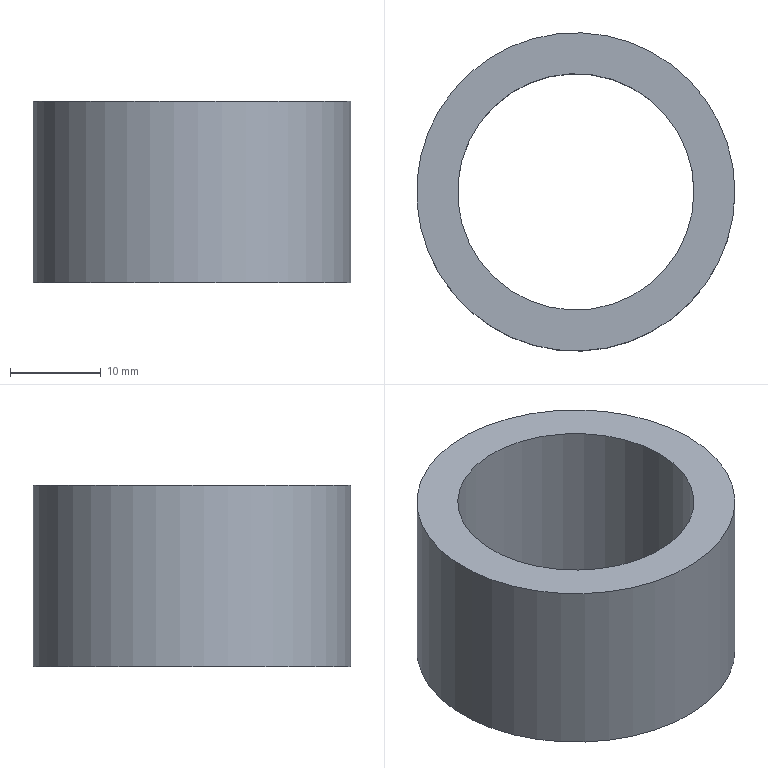Component | NX | BUSHING | 1 solid | 4 faces | box 35 x 35 x 20 mm | volume 8624 mm3 | cylinder 2 | plane 2 | commonest cylinder face diameters 35 x1 26 x1
STEP:
#1=CARTESIAN_POINT('',(0.,0.,0.));
#2=DIRECTION('',(0.,0.,1.));
#3=DIRECTION('',(1.,0.,0.));
#4=AXIS2_PLACEMENT_3D('',#1,#2,#3);
#5=CARTESIAN_POINT('',(30.5,0.,38.));
#6=VERTEX_POINT('',#5);
#7=CARTESIAN_POINT('',(13.,0.,38.));
#8=DIRECTION('',(0.,0.,1.));
#9=DIRECTION('',(1.,0.,0.));
#10=AXIS2_PLACEMENT_3D('',#7,#8,#9);
#11=CIRCLE('',#10,17.5);
#12=CARTESIAN_POINT('',(13.,0.,38.));
#13=DIRECTION('',(0.,0.,-1.));
#14=DIRECTION('',(-1.,0.,0.));
#15=AXIS2_PLACEMENT_3D('',#12,#13,#14);
#16=CYLINDRICAL_SURFACE('',#15,17.5);
#17=CARTESIAN_POINT('',(9.425,0.));
#18=DIRECTION('',(-1.,0.));
#19=VECTOR('',#18,1.);
#20=LINE('',#17,#19);
#21=(GEOMETRIC_REPRESENTATION_CONTEXT(2)PARAMETRIC_REPRESENTATION_CONTEXT()REPRESENTATION_CONTEXT('',''));
#22=DEFINITIONAL_REPRESENTATION('',(#20),#21);
#23=PCURVE('',#16,#22);
#24=CARTESIAN_POINT('',(13.,0.,38.));
#25=DIRECTION('',(0.,0.,1.));
#26=DIRECTION('',(1.,0.,0.));
#27=AXIS2_PLACEMENT_3D('',#24,#25,#26);
#28=PLANE('',#27);
#29=CARTESIAN_POINT('',(0.,0.));
#30=DIRECTION('',(1.,0.));
#31=AXIS2_PLACEMENT_2D('',#29,#30);
#32=CIRCLE('',#31,17.5);
#33=(GEOMETRIC_REPRESENTATION_CONTEXT(2)PARAMETRIC_REPRESENTATION_CONTEXT()REPRESENTATION_CONTEXT('',''));
#34=DEFINITIONAL_REPRESENTATION('',(#32),#33);
#35=PCURVE('',#28,#34);
#36=SURFACE_CURVE('',#11,(#23,#35),.PCURVE_S1.);
#37=EDGE_CURVE('',#6,#6,#36,.T.);
#38=ORIENTED_EDGE('',*,*,#37,.F.);
#39=CARTESIAN_POINT('',(30.5,0.,18.));
#40=VERTEX_POINT('',#39);
#41=CARTESIAN_POINT('',(30.5,0.,38.));
#42=CARTESIAN_POINT('',(30.5,0.,18.));
#43=B_SPLINE_CURVE_WITH_KNOTS('',1,(#41,#42),.UNSPECIFIED.,.F.,.F.,(2,2),(0.,20.),.PIECEWISE_BEZIER_KNOTS.);
#44=CARTESIAN_POINT('',(9.425,0.));
#45=DIRECTION('',(0.,1.));
#46=VECTOR('',#45,1.);
#47=LINE('',#44,#46);
#48=(GEOMETRIC_REPRESENTATION_CONTEXT(2)PARAMETRIC_REPRESENTATION_CONTEXT()REPRESENTATION_CONTEXT('',''));
#49=DEFINITIONAL_REPRESENTATION('',(#47),#48);
#50=PCURVE('',#16,#49);
#51=CARTESIAN_POINT('',(3.142,0.));
#52=DIRECTION('',(0.,1.));
#53=VECTOR('',#52,1.);
#54=LINE('',#51,#53);
#55=(GEOMETRIC_REPRESENTATION_CONTEXT(2)PARAMETRIC_REPRESENTATION_CONTEXT()REPRESENTATION_CONTEXT('',''));
#56=DEFINITIONAL_REPRESENTATION('',(#54),#55);
#57=PCURVE('',#16,#56);
#58=SEAM_CURVE('',#43,(#50,#57),.PCURVE_S1.);
#59=EDGE_CURVE('',#6,#40,#58,.T.);
#60=ORIENTED_EDGE('',*,*,#59,.T.);
#61=CARTESIAN_POINT('',(13.,0.,18.));
#62=DIRECTION('',(0.,0.,1.));
#63=DIRECTION('',(1.,0.,0.));
#64=AXIS2_PLACEMENT_3D('',#61,#62,#63);
#65=CIRCLE('',#64,17.5);
#66=CARTESIAN_POINT('',(9.425,20.));
#67=DIRECTION('',(-1.,0.));
#68=VECTOR('',#67,1.);
#69=LINE('',#66,#68);
#70=(GEOMETRIC_REPRESENTATION_CONTEXT(2)PARAMETRIC_REPRESENTATION_CONTEXT()REPRESENTATION_CONTEXT('',''));
#71=DEFINITIONAL_REPRESENTATION('',(#69),#70);
#72=PCURVE('',#16,#71);
#73=CARTESIAN_POINT('',(13.,0.,18.));
#74=DIRECTION('',(0.,0.,1.));
#75=DIRECTION('',(1.,0.,0.));
#76=AXIS2_PLACEMENT_3D('',#73,#74,#75);
#77=PLANE('',#76);
#78=CARTESIAN_POINT('',(0.,0.));
#79=DIRECTION('',(1.,0.));
#80=AXIS2_PLACEMENT_2D('',#78,#79);
#81=CIRCLE('',#80,17.5);
#82=(GEOMETRIC_REPRESENTATION_CONTEXT(2)PARAMETRIC_REPRESENTATION_CONTEXT()REPRESENTATION_CONTEXT('',''));
#83=DEFINITIONAL_REPRESENTATION('',(#81),#82);
#84=PCURVE('',#77,#83);
#85=SURFACE_CURVE('',#65,(#72,#84),.PCURVE_S1.);
#86=EDGE_CURVE('',#40,#40,#85,.T.);
#87=ORIENTED_EDGE('',*,*,#86,.T.);
#88=ORIENTED_EDGE('',*,*,#59,.F.);
#89=EDGE_LOOP('',(#38,#60,#87,#88));
#90=FACE_BOUND('',#89,.T.);
#91=ADVANCED_FACE('',(#90),#16,.T.);
#92=CARTESIAN_POINT('',(26.,0.,38.));
#93=VERTEX_POINT('',#92);
#94=CARTESIAN_POINT('',(13.,0.,38.));
#95=DIRECTION('',(0.,0.,1.));
#96=DIRECTION('',(1.,0.,0.));
#97=AXIS2_PLACEMENT_3D('',#94,#95,#96);
#98=CIRCLE('',#97,13.);
#99=CARTESIAN_POINT('',(13.,0.,38.));
#100=DIRECTION('',(0.,0.,-1.));
#101=DIRECTION('',(-1.,0.,0.));
#102=AXIS2_PLACEMENT_3D('',#99,#100,#101);
#103=CYLINDRICAL_SURFACE('',#102,13.);
#104=CARTESIAN_POINT('',(9.425,0.));
#105=DIRECTION('',(-1.,0.));
#106=VECTOR('',#105,1.);
#107=LINE('',#104,#106);
#108=(GEOMETRIC_REPRESENTATION_CONTEXT(2)PARAMETRIC_REPRESENTATION_CONTEXT()REPRESENTATION_CONTEXT('',''));
#109=DEFINITIONAL_REPRESENTATION('',(#107),#108);
#110=PCURVE('',#103,#109);
#111=CARTESIAN_POINT('',(0.,0.));
#112=DIRECTION('',(1.,0.));
#113=AXIS2_PLACEMENT_2D('',#111,#112);
#114=CIRCLE('',#113,13.);
#115=(GEOMETRIC_REPRESENTATION_CONTEXT(2)PARAMETRIC_REPRESENTATION_CONTEXT()REPRESENTATION_CONTEXT('',''));
#116=DEFINITIONAL_REPRESENTATION('',(#114),#115);
#117=PCURVE('',#28,#116);
#118=SURFACE_CURVE('',#98,(#110,#117),.PCURVE_S1.);
#119=EDGE_CURVE('',#93,#93,#118,.T.);
#120=ORIENTED_EDGE('',*,*,#119,.F.);
#121=CARTESIAN_POINT('',(26.,0.,18.));
#122=VERTEX_POINT('',#121);
#123=CARTESIAN_POINT('',(26.,0.,38.));
#124=CARTESIAN_POINT('',(26.,0.,18.));
#125=B_SPLINE_CURVE_WITH_KNOTS('',1,(#123,#124),.UNSPECIFIED.,.F.,.F.,(2,2),(0.,20.),.PIECEWISE_BEZIER_KNOTS.);
#126=CARTESIAN_POINT('',(9.425,0.));
#127=DIRECTION('',(0.,1.));
#128=VECTOR('',#127,1.);
#129=LINE('',#126,#128);
#130=(GEOMETRIC_REPRESENTATION_CONTEXT(2)PARAMETRIC_REPRESENTATION_CONTEXT()REPRESENTATION_CONTEXT('',''));
#131=DEFINITIONAL_REPRESENTATION('',(#129),#130);
#132=PCURVE('',#103,#131);
#133=CARTESIAN_POINT('',(3.142,0.));
#134=DIRECTION('',(0.,1.));
#135=VECTOR('',#134,1.);
#136=LINE('',#133,#135);
#137=(GEOMETRIC_REPRESENTATION_CONTEXT(2)PARAMETRIC_REPRESENTATION_CONTEXT()REPRESENTATION_CONTEXT('',''));
#138=DEFINITIONAL_REPRESENTATION('',(#136),#137);
#139=PCURVE('',#103,#138);
#140=SEAM_CURVE('',#125,(#132,#139),.PCURVE_S1.);
#141=EDGE_CURVE('',#93,#122,#140,.T.);
#142=ORIENTED_EDGE('',*,*,#141,.T.);
#143=CARTESIAN_POINT('',(13.,0.,18.));
#144=DIRECTION('',(0.,0.,1.));
#145=DIRECTION('',(1.,0.,0.));
#146=AXIS2_PLACEMENT_3D('',#143,#144,#145);
#147=CIRCLE('',#146,13.);
#148=CARTESIAN_POINT('',(9.425,20.));
#149=DIRECTION('',(-1.,0.));
#150=VECTOR('',#149,1.);
#151=LINE('',#148,#150);
#152=(GEOMETRIC_REPRESENTATION_CONTEXT(2)PARAMETRIC_REPRESENTATION_CONTEXT()REPRESENTATION_CONTEXT('',''));
#153=DEFINITIONAL_REPRESENTATION('',(#151),#152);
#154=PCURVE('',#103,#153);
#155=CARTESIAN_POINT('',(0.,0.));
#156=DIRECTION('',(1.,0.));
#157=AXIS2_PLACEMENT_2D('',#155,#156);
#158=CIRCLE('',#157,13.);
#159=(GEOMETRIC_REPRESENTATION_CONTEXT(2)PARAMETRIC_REPRESENTATION_CONTEXT()REPRESENTATION_CONTEXT('',''));
#160=DEFINITIONAL_REPRESENTATION('',(#158),#159);
#161=PCURVE('',#77,#160);
#162=SURFACE_CURVE('',#147,(#154,#161),.PCURVE_S1.);
#163=EDGE_CURVE('',#122,#122,#162,.T.);
#164=ORIENTED_EDGE('',*,*,#163,.T.);
#165=ORIENTED_EDGE('',*,*,#141,.F.);
#166=EDGE_LOOP('',(#120,#142,#164,#165));
#167=FACE_BOUND('',#166,.F.);
#168=ADVANCED_FACE('',(#167),#103,.F.);
#169=ORIENTED_EDGE('',*,*,#37,.T.);
#170=EDGE_LOOP('',(#169));
#171=FACE_BOUND('',#170,.T.);
#172=ORIENTED_EDGE('',*,*,#119,.F.);
#173=EDGE_LOOP('',(#172));
#174=FACE_BOUND('',#173,.T.);
#175=ADVANCED_FACE('',(#171,#174),#28,.T.);
#176=ORIENTED_EDGE('',*,*,#86,.F.);
#177=EDGE_LOOP('',(#176));
#178=FACE_BOUND('',#177,.T.);
#179=ORIENTED_EDGE('',*,*,#163,.T.);
#180=EDGE_LOOP('',(#179));
#181=FACE_BOUND('',#180,.T.);
#182=ADVANCED_FACE('',(#178,#181),#77,.F.);
#183=CLOSED_SHELL('',(#91,#168,#175,#182));
#184=MANIFOLD_SOLID_BREP('',#183);
#185=(LENGTH_UNIT()NAMED_UNIT(*)SI_UNIT(.MILLI.,.METRE.));
#186=UNCERTAINTY_MEASURE_WITH_UNIT(LENGTH_MEASURE(0.00001),#185,'','');
#187=(NAMED_UNIT(*)PLANE_ANGLE_UNIT()SI_UNIT($,.RADIAN.));
#188=(NAMED_UNIT(*)SI_UNIT($,.STERADIAN.)SOLID_ANGLE_UNIT());
#189=(GEOMETRIC_REPRESENTATION_CONTEXT(3)GLOBAL_UNCERTAINTY_ASSIGNED_CONTEXT((#186))GLOBAL_UNIT_ASSIGNED_CONTEXT((#185,#187,#188))REPRESENTATION_CONTEXT('',''));
#190=ADVANCED_BREP_SHAPE_REPRESENTATION('',(#4,#184),#189);